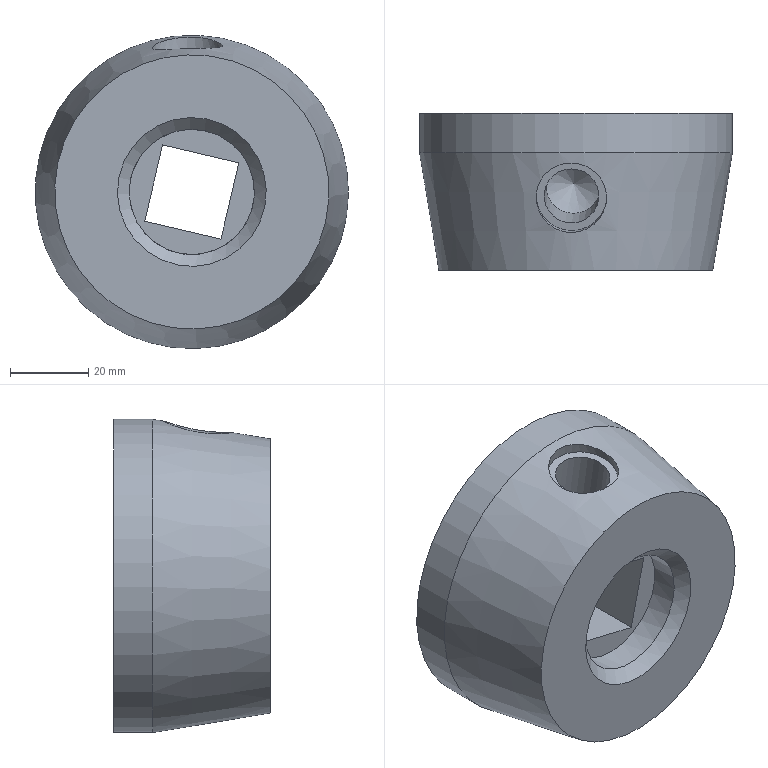Component | NX | TWIST_WHEEL | 1 solid | 15 faces | volume 159257 mm3 | plane 8 | cylinder 4 | cone 3 | commonest cylinder face diameters 80 x1 32 x1 18 x1 14 x1